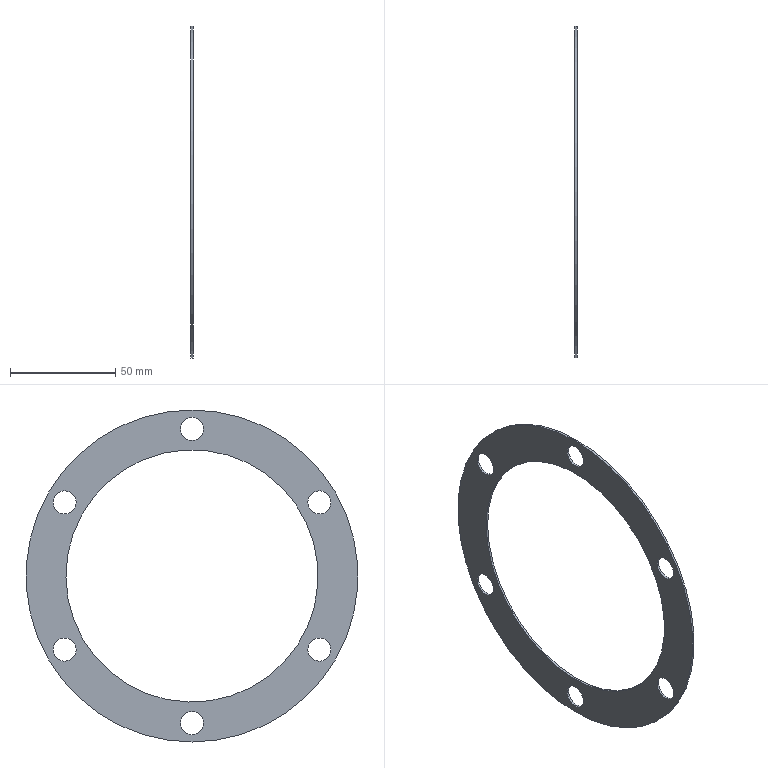Component | NX | T1_GASKET_2 | 1 solid | 10 faces | box 1 x 158 x 158 mm | volume 7727 mm3 | cylinder 8 | plane 2 | commonest cylinder face diameters 11 x6 120 x1 158 x1
STEP:
#1=CARTESIAN_POINT('',(0.,0.,0.));
#2=DIRECTION('',(0.,0.,1.));
#3=DIRECTION('',(1.,0.,0.));
#4=AXIS2_PLACEMENT_3D('',#1,#2,#3);
#5=CARTESIAN_POINT('',(279.,-0.,-78.5));
#6=VERTEX_POINT('',#5);
#7=CARTESIAN_POINT('',(279.,-0.,-73.));
#8=DIRECTION('',(1.,0.,0.));
#9=DIRECTION('',(0.,-0.,-1.));
#10=AXIS2_PLACEMENT_3D('',#7,#8,#9);
#11=CIRCLE('',#10,5.5);
#12=CARTESIAN_POINT('',(279.,-0.,-73.));
#13=DIRECTION('',(-1.,0.,0.));
#14=DIRECTION('',(0.,0.5,0.866));
#15=AXIS2_PLACEMENT_3D('',#12,#13,#14);
#16=CYLINDRICAL_SURFACE('',#15,5.5);
#17=CARTESIAN_POINT('',(8.901,0.));
#18=DIRECTION('',(-1.,0.));
#19=VECTOR('',#18,1.);
#20=LINE('',#17,#19);
#21=(GEOMETRIC_REPRESENTATION_CONTEXT(2)PARAMETRIC_REPRESENTATION_CONTEXT()REPRESENTATION_CONTEXT('',''));
#22=DEFINITIONAL_REPRESENTATION('',(#20),#21);
#23=PCURVE('',#16,#22);
#24=CARTESIAN_POINT('',(279.,30.311,14.5));
#25=DIRECTION('',(1.,0.,0.));
#26=DIRECTION('',(0.,-0.5,-0.866));
#27=AXIS2_PLACEMENT_3D('',#24,#25,#26);
#28=PLANE('',#27);
#29=CARTESIAN_POINT('',(90.933,17.5));
#30=DIRECTION('',(0.866,0.5));
#31=AXIS2_PLACEMENT_2D('',#29,#30);
#32=CIRCLE('',#31,5.5);
#33=(GEOMETRIC_REPRESENTATION_CONTEXT(2)PARAMETRIC_REPRESENTATION_CONTEXT()REPRESENTATION_CONTEXT('',''));
#34=DEFINITIONAL_REPRESENTATION('',(#32),#33);
#35=PCURVE('',#28,#34);
#36=SURFACE_CURVE('',#11,(#23,#35),.PCURVE_S1.);
#37=EDGE_CURVE('',#6,#6,#36,.T.);
#38=ORIENTED_EDGE('',*,*,#37,.F.);
#39=CARTESIAN_POINT('',(278.,-0.,-78.5));
#40=VERTEX_POINT('',#39);
#41=CARTESIAN_POINT('',(279.,-0.,-78.5));
#42=CARTESIAN_POINT('',(278.,-0.,-78.5));
#43=B_SPLINE_CURVE_WITH_KNOTS('',1,(#41,#42),.UNSPECIFIED.,.F.,.F.,(2,2),(0.,1.),.PIECEWISE_BEZIER_KNOTS.);
#44=CARTESIAN_POINT('',(8.901,0.));
#45=DIRECTION('',(0.,1.));
#46=VECTOR('',#45,1.);
#47=LINE('',#44,#46);
#48=(GEOMETRIC_REPRESENTATION_CONTEXT(2)PARAMETRIC_REPRESENTATION_CONTEXT()REPRESENTATION_CONTEXT('',''));
#49=DEFINITIONAL_REPRESENTATION('',(#47),#48);
#50=PCURVE('',#16,#49);
#51=CARTESIAN_POINT('',(2.618,0.));
#52=DIRECTION('',(0.,1.));
#53=VECTOR('',#52,1.);
#54=LINE('',#51,#53);
#55=(GEOMETRIC_REPRESENTATION_CONTEXT(2)PARAMETRIC_REPRESENTATION_CONTEXT()REPRESENTATION_CONTEXT('',''));
#56=DEFINITIONAL_REPRESENTATION('',(#54),#55);
#57=PCURVE('',#16,#56);
#58=SEAM_CURVE('',#43,(#50,#57),.PCURVE_S1.);
#59=EDGE_CURVE('',#6,#40,#58,.T.);
#60=ORIENTED_EDGE('',*,*,#59,.T.);
#61=CARTESIAN_POINT('',(278.,-0.,-73.));
#62=DIRECTION('',(1.,0.,0.));
#63=DIRECTION('',(0.,-0.,-1.));
#64=AXIS2_PLACEMENT_3D('',#61,#62,#63);
#65=CIRCLE('',#64,5.5);
#66=CARTESIAN_POINT('',(8.901,1.));
#67=DIRECTION('',(-1.,0.));
#68=VECTOR('',#67,1.);
#69=LINE('',#66,#68);
#70=(GEOMETRIC_REPRESENTATION_CONTEXT(2)PARAMETRIC_REPRESENTATION_CONTEXT()REPRESENTATION_CONTEXT('',''));
#71=DEFINITIONAL_REPRESENTATION('',(#69),#70);
#72=PCURVE('',#16,#71);
#73=CARTESIAN_POINT('',(278.,30.311,14.5));
#74=DIRECTION('',(1.,0.,0.));
#75=DIRECTION('',(0.,-0.5,-0.866));
#76=AXIS2_PLACEMENT_3D('',#73,#74,#75);
#77=PLANE('',#76);
#78=CARTESIAN_POINT('',(90.933,17.5));
#79=DIRECTION('',(0.866,0.5));
#80=AXIS2_PLACEMENT_2D('',#78,#79);
#81=CIRCLE('',#80,5.5);
#82=(GEOMETRIC_REPRESENTATION_CONTEXT(2)PARAMETRIC_REPRESENTATION_CONTEXT()REPRESENTATION_CONTEXT('',''));
#83=DEFINITIONAL_REPRESENTATION('',(#81),#82);
#84=PCURVE('',#77,#83);
#85=SURFACE_CURVE('',#65,(#72,#84),.PCURVE_S1.);
#86=EDGE_CURVE('',#40,#40,#85,.T.);
#87=ORIENTED_EDGE('',*,*,#86,.T.);
#88=ORIENTED_EDGE('',*,*,#59,.F.);
#89=EDGE_LOOP('',(#38,#60,#87,#88));
#90=FACE_BOUND('',#89,.F.);
#91=ADVANCED_FACE('',(#90),#16,.F.);
#92=CARTESIAN_POINT('',(279.,-65.385,-40.75));
#93=VERTEX_POINT('',#92);
#94=CARTESIAN_POINT('',(279.,-60.622,-38.));
#95=DIRECTION('',(1.,0.,0.));
#96=DIRECTION('',(0.,-0.866,-0.5));
#97=AXIS2_PLACEMENT_3D('',#94,#95,#96);
#98=CIRCLE('',#97,5.5);
#99=CARTESIAN_POINT('',(279.,-60.622,-38.));
#100=DIRECTION('',(-1.,0.,0.));
#101=DIRECTION('',(0.,0.5,0.866));
#102=AXIS2_PLACEMENT_3D('',#99,#100,#101);
#103=CYLINDRICAL_SURFACE('',#102,5.5);
#104=CARTESIAN_POINT('',(9.948,0.));
#105=DIRECTION('',(-1.,0.));
#106=VECTOR('',#105,1.);
#107=LINE('',#104,#106);
#108=(GEOMETRIC_REPRESENTATION_CONTEXT(2)PARAMETRIC_REPRESENTATION_CONTEXT()REPRESENTATION_CONTEXT('',''));
#109=DEFINITIONAL_REPRESENTATION('',(#107),#108);
#110=PCURVE('',#103,#109);
#111=CARTESIAN_POINT('',(90.933,-52.5));
#112=DIRECTION('',(0.866,-0.5));
#113=AXIS2_PLACEMENT_2D('',#111,#112);
#114=CIRCLE('',#113,5.5);
#115=(GEOMETRIC_REPRESENTATION_CONTEXT(2)PARAMETRIC_REPRESENTATION_CONTEXT()REPRESENTATION_CONTEXT('',''));
#116=DEFINITIONAL_REPRESENTATION('',(#114),#115);
#117=PCURVE('',#28,#116);
#118=SURFACE_CURVE('',#98,(#110,#117),.PCURVE_S1.);
#119=EDGE_CURVE('',#93,#93,#118,.T.);
#120=ORIENTED_EDGE('',*,*,#119,.F.);
#121=CARTESIAN_POINT('',(278.,-65.385,-40.75));
#122=VERTEX_POINT('',#121);
#123=CARTESIAN_POINT('',(279.,-65.385,-40.75));
#124=CARTESIAN_POINT('',(278.,-65.385,-40.75));
#125=B_SPLINE_CURVE_WITH_KNOTS('',1,(#123,#124),.UNSPECIFIED.,.F.,.F.,(2,2),(0.,1.),.PIECEWISE_BEZIER_KNOTS.);
#126=CARTESIAN_POINT('',(9.948,0.));
#127=DIRECTION('',(0.,1.));
#128=VECTOR('',#127,1.);
#129=LINE('',#126,#128);
#130=(GEOMETRIC_REPRESENTATION_CONTEXT(2)PARAMETRIC_REPRESENTATION_CONTEXT()REPRESENTATION_CONTEXT('',''));
#131=DEFINITIONAL_REPRESENTATION('',(#129),#130);
#132=PCURVE('',#103,#131);
#133=CARTESIAN_POINT('',(3.665,0.));
#134=DIRECTION('',(0.,1.));
#135=VECTOR('',#134,1.);
#136=LINE('',#133,#135);
#137=(GEOMETRIC_REPRESENTATION_CONTEXT(2)PARAMETRIC_REPRESENTATION_CONTEXT()REPRESENTATION_CONTEXT('',''));
#138=DEFINITIONAL_REPRESENTATION('',(#136),#137);
#139=PCURVE('',#103,#138);
#140=SEAM_CURVE('',#125,(#132,#139),.PCURVE_S1.);
#141=EDGE_CURVE('',#93,#122,#140,.T.);
#142=ORIENTED_EDGE('',*,*,#141,.T.);
#143=CARTESIAN_POINT('',(278.,-60.622,-38.));
#144=DIRECTION('',(1.,0.,0.));
#145=DIRECTION('',(0.,-0.866,-0.5));
#146=AXIS2_PLACEMENT_3D('',#143,#144,#145);
#147=CIRCLE('',#146,5.5);
#148=CARTESIAN_POINT('',(9.948,1.));
#149=DIRECTION('',(-1.,0.));
#150=VECTOR('',#149,1.);
#151=LINE('',#148,#150);
#152=(GEOMETRIC_REPRESENTATION_CONTEXT(2)PARAMETRIC_REPRESENTATION_CONTEXT()REPRESENTATION_CONTEXT('',''));
#153=DEFINITIONAL_REPRESENTATION('',(#151),#152);
#154=PCURVE('',#103,#153);
#155=CARTESIAN_POINT('',(90.933,-52.5));
#156=DIRECTION('',(0.866,-0.5));
#157=AXIS2_PLACEMENT_2D('',#155,#156);
#158=CIRCLE('',#157,5.5);
#159=(GEOMETRIC_REPRESENTATION_CONTEXT(2)PARAMETRIC_REPRESENTATION_CONTEXT()REPRESENTATION_CONTEXT('',''));
#160=DEFINITIONAL_REPRESENTATION('',(#158),#159);
#161=PCURVE('',#77,#160);
#162=SURFACE_CURVE('',#147,(#154,#161),.PCURVE_S1.);
#163=EDGE_CURVE('',#122,#122,#162,.T.);
#164=ORIENTED_EDGE('',*,*,#163,.T.);
#165=ORIENTED_EDGE('',*,*,#141,.F.);
#166=EDGE_LOOP('',(#120,#142,#164,#165));
#167=FACE_BOUND('',#166,.F.);
#168=ADVANCED_FACE('',(#167),#103,.F.);
#169=CARTESIAN_POINT('',(279.,-65.385,34.75));
#170=VERTEX_POINT('',#169);
#171=CARTESIAN_POINT('',(279.,-60.622,32.));
#172=DIRECTION('',(1.,0.,0.));
#173=DIRECTION('',(0.,-0.866,0.5));
#174=AXIS2_PLACEMENT_3D('',#171,#172,#173);
#175=CIRCLE('',#174,5.5);
#176=CARTESIAN_POINT('',(279.,-60.622,32.));
#177=DIRECTION('',(-1.,0.,0.));
#178=DIRECTION('',(0.,0.5,0.866));
#179=AXIS2_PLACEMENT_3D('',#176,#177,#178);
#180=CYLINDRICAL_SURFACE('',#179,5.5);
#181=CARTESIAN_POINT('',(10.996,0.));
#182=DIRECTION('',(-1.,0.));
#183=VECTOR('',#182,1.);
#184=LINE('',#181,#183);
#185=(GEOMETRIC_REPRESENTATION_CONTEXT(2)PARAMETRIC_REPRESENTATION_CONTEXT()REPRESENTATION_CONTEXT('',''));
#186=DEFINITIONAL_REPRESENTATION('',(#184),#185);
#187=PCURVE('',#180,#186);
#188=CARTESIAN_POINT('',(30.311,-87.5));
#189=DIRECTION('',(0.,-1.));
#190=AXIS2_PLACEMENT_2D('',#188,#189);
#191=CIRCLE('',#190,5.5);
#192=(GEOMETRIC_REPRESENTATION_CONTEXT(2)PARAMETRIC_REPRESENTATION_CONTEXT()REPRESENTATION_CONTEXT('',''));
#193=DEFINITIONAL_REPRESENTATION('',(#191),#192);
#194=PCURVE('',#28,#193);
#195=SURFACE_CURVE('',#175,(#187,#194),.PCURVE_S1.);
#196=EDGE_CURVE('',#170,#170,#195,.T.);
#197=ORIENTED_EDGE('',*,*,#196,.F.);
#198=CARTESIAN_POINT('',(278.,-65.385,34.75));
#199=VERTEX_POINT('',#198);
#200=CARTESIAN_POINT('',(279.,-65.385,34.75));
#201=CARTESIAN_POINT('',(278.,-65.385,34.75));
#202=B_SPLINE_CURVE_WITH_KNOTS('',1,(#200,#201),.UNSPECIFIED.,.F.,.F.,(2,2),(0.,1.),.PIECEWISE_BEZIER_KNOTS.);
#203=CARTESIAN_POINT('',(10.996,0.));
#204=DIRECTION('',(0.,1.));
#205=VECTOR('',#204,1.);
#206=LINE('',#203,#205);
#207=(GEOMETRIC_REPRESENTATION_CONTEXT(2)PARAMETRIC_REPRESENTATION_CONTEXT()REPRESENTATION_CONTEXT('',''));
#208=DEFINITIONAL_REPRESENTATION('',(#206),#207);
#209=PCURVE('',#180,#208);
#210=CARTESIAN_POINT('',(4.712,0.));
#211=DIRECTION('',(0.,1.));
#212=VECTOR('',#211,1.);
#213=LINE('',#210,#212);
#214=(GEOMETRIC_REPRESENTATION_CONTEXT(2)PARAMETRIC_REPRESENTATION_CONTEXT()REPRESENTATION_CONTEXT('',''));
#215=DEFINITIONAL_REPRESENTATION('',(#213),#214);
#216=PCURVE('',#180,#215);
#217=SEAM_CURVE('',#202,(#209,#216),.PCURVE_S1.);
#218=EDGE_CURVE('',#170,#199,#217,.T.);
#219=ORIENTED_EDGE('',*,*,#218,.T.);
#220=CARTESIAN_POINT('',(278.,-60.622,32.));
#221=DIRECTION('',(1.,0.,0.));
#222=DIRECTION('',(0.,-0.866,0.5));
#223=AXIS2_PLACEMENT_3D('',#220,#221,#222);
#224=CIRCLE('',#223,5.5);
#225=CARTESIAN_POINT('',(10.996,1.));
#226=DIRECTION('',(-1.,0.));
#227=VECTOR('',#226,1.);
#228=LINE('',#225,#227);
#229=(GEOMETRIC_REPRESENTATION_CONTEXT(2)PARAMETRIC_REPRESENTATION_CONTEXT()REPRESENTATION_CONTEXT('',''));
#230=DEFINITIONAL_REPRESENTATION('',(#228),#229);
#231=PCURVE('',#180,#230);
#232=CARTESIAN_POINT('',(30.311,-87.5));
#233=DIRECTION('',(0.,-1.));
#234=AXIS2_PLACEMENT_2D('',#232,#233);
#235=CIRCLE('',#234,5.5);
#236=(GEOMETRIC_REPRESENTATION_CONTEXT(2)PARAMETRIC_REPRESENTATION_CONTEXT()REPRESENTATION_CONTEXT('',''));
#237=DEFINITIONAL_REPRESENTATION('',(#235),#236);
#238=PCURVE('',#77,#237);
#239=SURFACE_CURVE('',#224,(#231,#238),.PCURVE_S1.);
#240=EDGE_CURVE('',#199,#199,#239,.T.);
#241=ORIENTED_EDGE('',*,*,#240,.T.);
#242=ORIENTED_EDGE('',*,*,#218,.F.);
#243=EDGE_LOOP('',(#197,#219,#241,#242));
#244=FACE_BOUND('',#243,.F.);
#245=ADVANCED_FACE('',(#244),#180,.F.);
#246=CARTESIAN_POINT('',(279.,51.962,-33.));
#247=VERTEX_POINT('',#246);
#248=CARTESIAN_POINT('',(279.,0.,-3.));
#249=DIRECTION('',(1.,0.,0.));
#250=DIRECTION('',(0.,0.866,-0.5));
#251=AXIS2_PLACEMENT_3D('',#248,#249,#250);
#252=CIRCLE('',#251,60.);
#253=CARTESIAN_POINT('',(279.,0.,-3.));
#254=DIRECTION('',(-1.,0.,0.));
#255=DIRECTION('',(0.,0.5,0.866));
#256=AXIS2_PLACEMENT_3D('',#253,#254,#255);
#257=CYLINDRICAL_SURFACE('',#256,60.);
#258=CARTESIAN_POINT('',(7.854,0.));
#259=DIRECTION('',(-1.,0.));
#260=VECTOR('',#259,1.);
#261=LINE('',#258,#260);
#262=(GEOMETRIC_REPRESENTATION_CONTEXT(2)PARAMETRIC_REPRESENTATION_CONTEXT()REPRESENTATION_CONTEXT('',''));
#263=DEFINITIONAL_REPRESENTATION('',(#261),#262);
#264=PCURVE('',#257,#263);
#265=CARTESIAN_POINT('',(30.311,-17.5));
#266=DIRECTION('',(0.,1.));
#267=AXIS2_PLACEMENT_2D('',#265,#266);
#268=CIRCLE('',#267,60.);
#269=(GEOMETRIC_REPRESENTATION_CONTEXT(2)PARAMETRIC_REPRESENTATION_CONTEXT()REPRESENTATION_CONTEXT('',''));
#270=DEFINITIONAL_REPRESENTATION('',(#268),#269);
#271=PCURVE('',#28,#270);
#272=SURFACE_CURVE('',#252,(#264,#271),.PCURVE_S1.);
#273=EDGE_CURVE('',#247,#247,#272,.T.);
#274=ORIENTED_EDGE('',*,*,#273,.F.);
#275=CARTESIAN_POINT('',(278.,51.962,-33.));
#276=VERTEX_POINT('',#275);
#277=CARTESIAN_POINT('',(279.,51.962,-33.));
#278=CARTESIAN_POINT('',(278.,51.962,-33.));
#279=B_SPLINE_CURVE_WITH_KNOTS('',1,(#277,#278),.UNSPECIFIED.,.F.,.F.,(2,2),(0.,1.),.PIECEWISE_BEZIER_KNOTS.);
#280=CARTESIAN_POINT('',(7.854,0.));
#281=DIRECTION('',(0.,1.));
#282=VECTOR('',#281,1.);
#283=LINE('',#280,#282);
#284=(GEOMETRIC_REPRESENTATION_CONTEXT(2)PARAMETRIC_REPRESENTATION_CONTEXT()REPRESENTATION_CONTEXT('',''));
#285=DEFINITIONAL_REPRESENTATION('',(#283),#284);
#286=PCURVE('',#257,#285);
#287=CARTESIAN_POINT('',(1.571,0.));
#288=DIRECTION('',(0.,1.));
#289=VECTOR('',#288,1.);
#290=LINE('',#287,#289);
#291=(GEOMETRIC_REPRESENTATION_CONTEXT(2)PARAMETRIC_REPRESENTATION_CONTEXT()REPRESENTATION_CONTEXT('',''));
#292=DEFINITIONAL_REPRESENTATION('',(#290),#291);
#293=PCURVE('',#257,#292);
#294=SEAM_CURVE('',#279,(#286,#293),.PCURVE_S1.);
#295=EDGE_CURVE('',#247,#276,#294,.T.);
#296=ORIENTED_EDGE('',*,*,#295,.T.);
#297=CARTESIAN_POINT('',(278.,0.,-3.));
#298=DIRECTION('',(1.,0.,0.));
#299=DIRECTION('',(0.,0.866,-0.5));
#300=AXIS2_PLACEMENT_3D('',#297,#298,#299);
#301=CIRCLE('',#300,60.);
#302=CARTESIAN_POINT('',(7.854,1.));
#303=DIRECTION('',(-1.,0.));
#304=VECTOR('',#303,1.);
#305=LINE('',#302,#304);
#306=(GEOMETRIC_REPRESENTATION_CONTEXT(2)PARAMETRIC_REPRESENTATION_CONTEXT()REPRESENTATION_CONTEXT('',''));
#307=DEFINITIONAL_REPRESENTATION('',(#305),#306);
#308=PCURVE('',#257,#307);
#309=CARTESIAN_POINT('',(30.311,-17.5));
#310=DIRECTION('',(0.,1.));
#311=AXIS2_PLACEMENT_2D('',#309,#310);
#312=CIRCLE('',#311,60.);
#313=(GEOMETRIC_REPRESENTATION_CONTEXT(2)PARAMETRIC_REPRESENTATION_CONTEXT()REPRESENTATION_CONTEXT('',''));
#314=DEFINITIONAL_REPRESENTATION('',(#312),#313);
#315=PCURVE('',#77,#314);
#316=SURFACE_CURVE('',#301,(#308,#315),.PCURVE_S1.);
#317=EDGE_CURVE('',#276,#276,#316,.T.);
#318=ORIENTED_EDGE('',*,*,#317,.T.);
#319=ORIENTED_EDGE('',*,*,#295,.F.);
#320=EDGE_LOOP('',(#274,#296,#318,#319));
#321=FACE_BOUND('',#320,.F.);
#322=ADVANCED_FACE('',(#321),#257,.F.);
#323=CARTESIAN_POINT('',(279.,0.,72.5));
#324=VERTEX_POINT('',#323);
#325=CARTESIAN_POINT('',(279.,0.,67.));
#326=DIRECTION('',(1.,0.,0.));
#327=DIRECTION('',(0.,0.,1.));
#328=AXIS2_PLACEMENT_3D('',#325,#326,#327);
#329=CIRCLE('',#328,5.5);
#330=CARTESIAN_POINT('',(279.,0.,67.));
#331=DIRECTION('',(-1.,0.,0.));
#332=DIRECTION('',(0.,0.5,0.866));
#333=AXIS2_PLACEMENT_3D('',#330,#331,#332);
#334=CYLINDRICAL_SURFACE('',#333,5.5);
#335=CARTESIAN_POINT('',(12.043,0.));
#336=DIRECTION('',(-1.,0.));
#337=VECTOR('',#336,1.);
#338=LINE('',#335,#337);
#339=(GEOMETRIC_REPRESENTATION_CONTEXT(2)PARAMETRIC_REPRESENTATION_CONTEXT()REPRESENTATION_CONTEXT('',''));
#340=DEFINITIONAL_REPRESENTATION('',(#338),#339);
#341=PCURVE('',#334,#340);
#342=CARTESIAN_POINT('',(-30.311,-52.5));
#343=DIRECTION('',(-0.866,-0.5));
#344=AXIS2_PLACEMENT_2D('',#342,#343);
#345=CIRCLE('',#344,5.5);
#346=(GEOMETRIC_REPRESENTATION_CONTEXT(2)PARAMETRIC_REPRESENTATION_CONTEXT()REPRESENTATION_CONTEXT('',''));
#347=DEFINITIONAL_REPRESENTATION('',(#345),#346);
#348=PCURVE('',#28,#347);
#349=SURFACE_CURVE('',#329,(#341,#348),.PCURVE_S1.);
#350=EDGE_CURVE('',#324,#324,#349,.T.);
#351=ORIENTED_EDGE('',*,*,#350,.F.);
#352=CARTESIAN_POINT('',(278.,0.,72.5));
#353=VERTEX_POINT('',#352);
#354=CARTESIAN_POINT('',(279.,0.,72.5));
#355=CARTESIAN_POINT('',(278.,0.,72.5));
#356=B_SPLINE_CURVE_WITH_KNOTS('',1,(#354,#355),.UNSPECIFIED.,.F.,.F.,(2,2),(0.,1.),.PIECEWISE_BEZIER_KNOTS.);
#357=CARTESIAN_POINT('',(12.043,0.));
#358=DIRECTION('',(0.,1.));
#359=VECTOR('',#358,1.);
#360=LINE('',#357,#359);
#361=(GEOMETRIC_REPRESENTATION_CONTEXT(2)PARAMETRIC_REPRESENTATION_CONTEXT()REPRESENTATION_CONTEXT('',''));
#362=DEFINITIONAL_REPRESENTATION('',(#360),#361);
#363=PCURVE('',#334,#362);
#364=CARTESIAN_POINT('',(5.76,0.));
#365=DIRECTION('',(0.,1.));
#366=VECTOR('',#365,1.);
#367=LINE('',#364,#366);
#368=(GEOMETRIC_REPRESENTATION_CONTEXT(2)PARAMETRIC_REPRESENTATION_CONTEXT()REPRESENTATION_CONTEXT('',''));
#369=DEFINITIONAL_REPRESENTATION('',(#367),#368);
#370=PCURVE('',#334,#369);
#371=SEAM_CURVE('',#356,(#363,#370),.PCURVE_S1.);
#372=EDGE_CURVE('',#324,#353,#371,.T.);
#373=ORIENTED_EDGE('',*,*,#372,.T.);
#374=CARTESIAN_POINT('',(278.,0.,67.));
#375=DIRECTION('',(1.,0.,0.));
#376=DIRECTION('',(0.,0.,1.));
#377=AXIS2_PLACEMENT_3D('',#374,#375,#376);
#378=CIRCLE('',#377,5.5);
#379=CARTESIAN_POINT('',(12.043,1.));
#380=DIRECTION('',(-1.,0.));
#381=VECTOR('',#380,1.);
#382=LINE('',#379,#381);
#383=(GEOMETRIC_REPRESENTATION_CONTEXT(2)PARAMETRIC_REPRESENTATION_CONTEXT()REPRESENTATION_CONTEXT('',''));
#384=DEFINITIONAL_REPRESENTATION('',(#382),#383);
#385=PCURVE('',#334,#384);
#386=CARTESIAN_POINT('',(-30.311,-52.5));
#387=DIRECTION('',(-0.866,-0.5));
#388=AXIS2_PLACEMENT_2D('',#386,#387);
#389=CIRCLE('',#388,5.5);
#390=(GEOMETRIC_REPRESENTATION_CONTEXT(2)PARAMETRIC_REPRESENTATION_CONTEXT()REPRESENTATION_CONTEXT('',''));
#391=DEFINITIONAL_REPRESENTATION('',(#389),#390);
#392=PCURVE('',#77,#391);
#393=SURFACE_CURVE('',#378,(#385,#392),.PCURVE_S1.);
#394=EDGE_CURVE('',#353,#353,#393,.T.);
#395=ORIENTED_EDGE('',*,*,#394,.T.);
#396=ORIENTED_EDGE('',*,*,#372,.F.);
#397=EDGE_LOOP('',(#351,#373,#395,#396));
#398=FACE_BOUND('',#397,.F.);
#399=ADVANCED_FACE('',(#398),#334,.F.);
#400=CARTESIAN_POINT('',(279.,65.385,34.75));
#401=VERTEX_POINT('',#400);
#402=CARTESIAN_POINT('',(279.,60.622,32.));
#403=DIRECTION('',(1.,0.,0.));
#404=DIRECTION('',(0.,0.866,0.5));
#405=AXIS2_PLACEMENT_3D('',#402,#403,#404);
#406=CIRCLE('',#405,5.5);
#407=CARTESIAN_POINT('',(279.,60.622,32.));
#408=DIRECTION('',(-1.,0.,0.));
#409=DIRECTION('',(0.,0.5,0.866));
#410=AXIS2_PLACEMENT_3D('',#407,#408,#409);
#411=CYLINDRICAL_SURFACE('',#410,5.5);
#412=CARTESIAN_POINT('',(6.807,0.));
#413=DIRECTION('',(-1.,0.));
#414=VECTOR('',#413,1.);
#415=LINE('',#412,#414);
#416=(GEOMETRIC_REPRESENTATION_CONTEXT(2)PARAMETRIC_REPRESENTATION_CONTEXT()REPRESENTATION_CONTEXT('',''));
#417=DEFINITIONAL_REPRESENTATION('',(#415),#416);
#418=PCURVE('',#411,#417);
#419=CARTESIAN_POINT('',(-30.311,17.5));
#420=DIRECTION('',(-0.866,0.5));
#421=AXIS2_PLACEMENT_2D('',#419,#420);
#422=CIRCLE('',#421,5.5);
#423=(GEOMETRIC_REPRESENTATION_CONTEXT(2)PARAMETRIC_REPRESENTATION_CONTEXT()REPRESENTATION_CONTEXT('',''));
#424=DEFINITIONAL_REPRESENTATION('',(#422),#423);
#425=PCURVE('',#28,#424);
#426=SURFACE_CURVE('',#406,(#418,#425),.PCURVE_S1.);
#427=EDGE_CURVE('',#401,#401,#426,.T.);
#428=ORIENTED_EDGE('',*,*,#427,.F.);
#429=CARTESIAN_POINT('',(278.,65.385,34.75));
#430=VERTEX_POINT('',#429);
#431=CARTESIAN_POINT('',(279.,65.385,34.75));
#432=CARTESIAN_POINT('',(278.,65.385,34.75));
#433=B_SPLINE_CURVE_WITH_KNOTS('',1,(#431,#432),.UNSPECIFIED.,.F.,.F.,(2,2),(0.,1.),.PIECEWISE_BEZIER_KNOTS.);
#434=CARTESIAN_POINT('',(6.807,0.));
#435=DIRECTION('',(0.,1.));
#436=VECTOR('',#435,1.);
#437=LINE('',#434,#436);
#438=(GEOMETRIC_REPRESENTATION_CONTEXT(2)PARAMETRIC_REPRESENTATION_CONTEXT()REPRESENTATION_CONTEXT('',''));
#439=DEFINITIONAL_REPRESENTATION('',(#437),#438);
#440=PCURVE('',#411,#439);
#441=CARTESIAN_POINT('',(0.5236,0.));
#442=DIRECTION('',(0.,1.));
#443=VECTOR('',#442,1.);
#444=LINE('',#441,#443);
#445=(GEOMETRIC_REPRESENTATION_CONTEXT(2)PARAMETRIC_REPRESENTATION_CONTEXT()REPRESENTATION_CONTEXT('',''));
#446=DEFINITIONAL_REPRESENTATION('',(#444),#445);
#447=PCURVE('',#411,#446);
#448=SEAM_CURVE('',#433,(#440,#447),.PCURVE_S1.);
#449=EDGE_CURVE('',#401,#430,#448,.T.);
#450=ORIENTED_EDGE('',*,*,#449,.T.);
#451=CARTESIAN_POINT('',(278.,60.622,32.));
#452=DIRECTION('',(1.,0.,0.));
#453=DIRECTION('',(0.,0.866,0.5));
#454=AXIS2_PLACEMENT_3D('',#451,#452,#453);
#455=CIRCLE('',#454,5.5);
#456=CARTESIAN_POINT('',(6.807,1.));
#457=DIRECTION('',(-1.,0.));
#458=VECTOR('',#457,1.);
#459=LINE('',#456,#458);
#460=(GEOMETRIC_REPRESENTATION_CONTEXT(2)PARAMETRIC_REPRESENTATION_CONTEXT()REPRESENTATION_CONTEXT('',''));
#461=DEFINITIONAL_REPRESENTATION('',(#459),#460);
#462=PCURVE('',#411,#461);
#463=CARTESIAN_POINT('',(-30.311,17.5));
#464=DIRECTION('',(-0.866,0.5));
#465=AXIS2_PLACEMENT_2D('',#463,#464);
#466=CIRCLE('',#465,5.5);
#467=(GEOMETRIC_REPRESENTATION_CONTEXT(2)PARAMETRIC_REPRESENTATION_CONTEXT()REPRESENTATION_CONTEXT('',''));
#468=DEFINITIONAL_REPRESENTATION('',(#466),#467);
#469=PCURVE('',#77,#468);
#470=SURFACE_CURVE('',#455,(#462,#469),.PCURVE_S1.);
#471=EDGE_CURVE('',#430,#430,#470,.T.);
#472=ORIENTED_EDGE('',*,*,#471,.T.);
#473=ORIENTED_EDGE('',*,*,#449,.F.);
#474=EDGE_LOOP('',(#428,#450,#472,#473));
#475=FACE_BOUND('',#474,.F.);
#476=ADVANCED_FACE('',(#475),#411,.F.);
#477=CARTESIAN_POINT('',(279.,68.416,-42.5));
#478=VERTEX_POINT('',#477);
#479=CARTESIAN_POINT('',(279.,0.,-3.));
#480=DIRECTION('',(1.,0.,0.));
#481=DIRECTION('',(0.,0.866,-0.5));
#482=AXIS2_PLACEMENT_3D('',#479,#480,#481);
#483=CIRCLE('',#482,79.);
#484=CARTESIAN_POINT('',(279.,0.,-3.));
#485=DIRECTION('',(-1.,0.,0.));
#486=DIRECTION('',(0.,0.5,0.866));
#487=AXIS2_PLACEMENT_3D('',#484,#485,#486);
#488=CYLINDRICAL_SURFACE('',#487,79.);
#489=CARTESIAN_POINT('',(7.854,0.));
#490=DIRECTION('',(-1.,0.));
#491=VECTOR('',#490,1.);
#492=LINE('',#489,#491);
#493=(GEOMETRIC_REPRESENTATION_CONTEXT(2)PARAMETRIC_REPRESENTATION_CONTEXT()REPRESENTATION_CONTEXT('',''));
#494=DEFINITIONAL_REPRESENTATION('',(#492),#493);
#495=PCURVE('',#488,#494);
#496=CARTESIAN_POINT('',(30.311,-17.5));
#497=DIRECTION('',(0.,1.));
#498=AXIS2_PLACEMENT_2D('',#496,#497);
#499=CIRCLE('',#498,79.);
#500=(GEOMETRIC_REPRESENTATION_CONTEXT(2)PARAMETRIC_REPRESENTATION_CONTEXT()REPRESENTATION_CONTEXT('',''));
#501=DEFINITIONAL_REPRESENTATION('',(#499),#500);
#502=PCURVE('',#28,#501);
#503=SURFACE_CURVE('',#483,(#495,#502),.PCURVE_S1.);
#504=EDGE_CURVE('',#478,#478,#503,.T.);
#505=ORIENTED_EDGE('',*,*,#504,.F.);
#506=CARTESIAN_POINT('',(278.,68.416,-42.5));
#507=VERTEX_POINT('',#506);
#508=CARTESIAN_POINT('',(279.,68.416,-42.5));
#509=CARTESIAN_POINT('',(278.,68.416,-42.5));
#510=B_SPLINE_CURVE_WITH_KNOTS('',1,(#508,#509),.UNSPECIFIED.,.F.,.F.,(2,2),(0.,1.),.PIECEWISE_BEZIER_KNOTS.);
#511=CARTESIAN_POINT('',(7.854,0.));
#512=DIRECTION('',(0.,1.));
#513=VECTOR('',#512,1.);
#514=LINE('',#511,#513);
#515=(GEOMETRIC_REPRESENTATION_CONTEXT(2)PARAMETRIC_REPRESENTATION_CONTEXT()REPRESENTATION_CONTEXT('',''));
#516=DEFINITIONAL_REPRESENTATION('',(#514),#515);
#517=PCURVE('',#488,#516);
#518=CARTESIAN_POINT('',(1.571,0.));
#519=DIRECTION('',(0.,1.));
#520=VECTOR('',#519,1.);
#521=LINE('',#518,#520);
#522=(GEOMETRIC_REPRESENTATION_CONTEXT(2)PARAMETRIC_REPRESENTATION_CONTEXT()REPRESENTATION_CONTEXT('',''));
#523=DEFINITIONAL_REPRESENTATION('',(#521),#522);
#524=PCURVE('',#488,#523);
#525=SEAM_CURVE('',#510,(#517,#524),.PCURVE_S1.);
#526=EDGE_CURVE('',#478,#507,#525,.T.);
#527=ORIENTED_EDGE('',*,*,#526,.T.);
#528=CARTESIAN_POINT('',(278.,0.,-3.));
#529=DIRECTION('',(1.,0.,0.));
#530=DIRECTION('',(0.,0.866,-0.5));
#531=AXIS2_PLACEMENT_3D('',#528,#529,#530);
#532=CIRCLE('',#531,79.);
#533=CARTESIAN_POINT('',(7.854,1.));
#534=DIRECTION('',(-1.,0.));
#535=VECTOR('',#534,1.);
#536=LINE('',#533,#535);
#537=(GEOMETRIC_REPRESENTATION_CONTEXT(2)PARAMETRIC_REPRESENTATION_CONTEXT()REPRESENTATION_CONTEXT('',''));
#538=DEFINITIONAL_REPRESENTATION('',(#536),#537);
#539=PCURVE('',#488,#538);
#540=CARTESIAN_POINT('',(30.311,-17.5));
#541=DIRECTION('',(0.,1.));
#542=AXIS2_PLACEMENT_2D('',#540,#541);
#543=CIRCLE('',#542,79.);
#544=(GEOMETRIC_REPRESENTATION_CONTEXT(2)PARAMETRIC_REPRESENTATION_CONTEXT()REPRESENTATION_CONTEXT('',''));
#545=DEFINITIONAL_REPRESENTATION('',(#543),#544);
#546=PCURVE('',#77,#545);
#547=SURFACE_CURVE('',#532,(#539,#546),.PCURVE_S1.);
#548=EDGE_CURVE('',#507,#507,#547,.T.);
#549=ORIENTED_EDGE('',*,*,#548,.T.);
#550=ORIENTED_EDGE('',*,*,#526,.F.);
#551=EDGE_LOOP('',(#505,#527,#549,#550));
#552=FACE_BOUND('',#551,.T.);
#553=ADVANCED_FACE('',(#552),#488,.T.);
#554=CARTESIAN_POINT('',(279.,65.385,-40.75));
#555=VERTEX_POINT('',#554);
#556=CARTESIAN_POINT('',(279.,60.622,-38.));
#557=DIRECTION('',(1.,0.,0.));
#558=DIRECTION('',(0.,0.866,-0.5));
#559=AXIS2_PLACEMENT_3D('',#556,#557,#558);
#560=CIRCLE('',#559,5.5);
#561=CARTESIAN_POINT('',(279.,60.622,-38.));
#562=DIRECTION('',(-1.,0.,0.));
#563=DIRECTION('',(0.,0.5,0.866));
#564=AXIS2_PLACEMENT_3D('',#561,#562,#563);
#565=CYLINDRICAL_SURFACE('',#564,5.5);
#566=CARTESIAN_POINT('',(7.854,0.));
#567=DIRECTION('',(-1.,0.));
#568=VECTOR('',#567,1.);
#569=LINE('',#566,#568);
#570=(GEOMETRIC_REPRESENTATION_CONTEXT(2)PARAMETRIC_REPRESENTATION_CONTEXT()REPRESENTATION_CONTEXT('',''));
#571=DEFINITIONAL_REPRESENTATION('',(#569),#570);
#572=PCURVE('',#565,#571);
#573=CARTESIAN_POINT('',(30.311,52.5));
#574=DIRECTION('',(-0.,1.));
#575=AXIS2_PLACEMENT_2D('',#573,#574);
#576=CIRCLE('',#575,5.5);
#577=(GEOMETRIC_REPRESENTATION_CONTEXT(2)PARAMETRIC_REPRESENTATION_CONTEXT()REPRESENTATION_CONTEXT('',''));
#578=DEFINITIONAL_REPRESENTATION('',(#576),#577);
#579=PCURVE('',#28,#578);
#580=SURFACE_CURVE('',#560,(#572,#579),.PCURVE_S1.);
#581=EDGE_CURVE('',#555,#555,#580,.T.);
#582=ORIENTED_EDGE('',*,*,#581,.F.);
#583=CARTESIAN_POINT('',(278.,65.385,-40.75));
#584=VERTEX_POINT('',#583);
#585=CARTESIAN_POINT('',(279.,65.385,-40.75));
#586=CARTESIAN_POINT('',(278.,65.385,-40.75));
#587=B_SPLINE_CURVE_WITH_KNOTS('',1,(#585,#586),.UNSPECIFIED.,.F.,.F.,(2,2),(0.,1.),.PIECEWISE_BEZIER_KNOTS.);
#588=CARTESIAN_POINT('',(7.854,0.));
#589=DIRECTION('',(0.,1.));
#590=VECTOR('',#589,1.);
#591=LINE('',#588,#590);
#592=(GEOMETRIC_REPRESENTATION_CONTEXT(2)PARAMETRIC_REPRESENTATION_CONTEXT()REPRESENTATION_CONTEXT('',''));
#593=DEFINITIONAL_REPRESENTATION('',(#591),#592);
#594=PCURVE('',#565,#593);
#595=CARTESIAN_POINT('',(1.571,0.));
#596=DIRECTION('',(0.,1.));
#597=VECTOR('',#596,1.);
#598=LINE('',#595,#597);
#599=(GEOMETRIC_REPRESENTATION_CONTEXT(2)PARAMETRIC_REPRESENTATION_CONTEXT()REPRESENTATION_CONTEXT('',''));
#600=DEFINITIONAL_REPRESENTATION('',(#598),#599);
#601=PCURVE('',#565,#600);
#602=SEAM_CURVE('',#587,(#594,#601),.PCURVE_S1.);
#603=EDGE_CURVE('',#555,#584,#602,.T.);
#604=ORIENTED_EDGE('',*,*,#603,.T.);
#605=CARTESIAN_POINT('',(278.,60.622,-38.));
#606=DIRECTION('',(1.,0.,0.));
#607=DIRECTION('',(0.,0.866,-0.5));
#608=AXIS2_PLACEMENT_3D('',#605,#606,#607);
#609=CIRCLE('',#608,5.5);
#610=CARTESIAN_POINT('',(7.854,1.));
#611=DIRECTION('',(-1.,0.));
#612=VECTOR('',#611,1.);
#613=LINE('',#610,#612);
#614=(GEOMETRIC_REPRESENTATION_CONTEXT(2)PARAMETRIC_REPRESENTATION_CONTEXT()REPRESENTATION_CONTEXT('',''));
#615=DEFINITIONAL_REPRESENTATION('',(#613),#614);
#616=PCURVE('',#565,#615);
#617=CARTESIAN_POINT('',(30.311,52.5));
#618=DIRECTION('',(-0.,1.));
#619=AXIS2_PLACEMENT_2D('',#617,#618);
#620=CIRCLE('',#619,5.5);
#621=(GEOMETRIC_REPRESENTATION_CONTEXT(2)PARAMETRIC_REPRESENTATION_CONTEXT()REPRESENTATION_CONTEXT('',''));
#622=DEFINITIONAL_REPRESENTATION('',(#620),#621);
#623=PCURVE('',#77,#622);
#624=SURFACE_CURVE('',#609,(#616,#623),.PCURVE_S1.);
#625=EDGE_CURVE('',#584,#584,#624,.T.);
#626=ORIENTED_EDGE('',*,*,#625,.T.);
#627=ORIENTED_EDGE('',*,*,#603,.F.);
#628=EDGE_LOOP('',(#582,#604,#626,#627));
#629=FACE_BOUND('',#628,.F.);
#630=ADVANCED_FACE('',(#629),#565,.F.);
#631=ORIENTED_EDGE('',*,*,#504,.T.);
#632=EDGE_LOOP('',(#631));
#633=FACE_BOUND('',#632,.T.);
#634=ORIENTED_EDGE('',*,*,#427,.F.);
#635=EDGE_LOOP('',(#634));
#636=FACE_BOUND('',#635,.T.);
#637=ORIENTED_EDGE('',*,*,#350,.F.);
#638=EDGE_LOOP('',(#637));
#639=FACE_BOUND('',#638,.T.);
#640=ORIENTED_EDGE('',*,*,#273,.F.);
#641=EDGE_LOOP('',(#640));
#642=FACE_BOUND('',#641,.T.);
#643=ORIENTED_EDGE('',*,*,#196,.F.);
#644=EDGE_LOOP('',(#643));
#645=FACE_BOUND('',#644,.T.);
#646=ORIENTED_EDGE('',*,*,#119,.F.);
#647=EDGE_LOOP('',(#646));
#648=FACE_BOUND('',#647,.T.);
#649=ORIENTED_EDGE('',*,*,#37,.F.);
#650=EDGE_LOOP('',(#649));
#651=FACE_BOUND('',#650,.T.);
#652=ORIENTED_EDGE('',*,*,#581,.F.);
#653=EDGE_LOOP('',(#652));
#654=FACE_BOUND('',#653,.T.);
#655=ADVANCED_FACE('',(#633,#636,#639,#642,#645,#648,#651,#654),#28,.T.);
#656=ORIENTED_EDGE('',*,*,#548,.F.);
#657=EDGE_LOOP('',(#656));
#658=FACE_BOUND('',#657,.T.);
#659=ORIENTED_EDGE('',*,*,#471,.T.);
#660=EDGE_LOOP('',(#659));
#661=FACE_BOUND('',#660,.T.);
#662=ORIENTED_EDGE('',*,*,#394,.T.);
#663=EDGE_LOOP('',(#662));
#664=FACE_BOUND('',#663,.T.);
#665=ORIENTED_EDGE('',*,*,#317,.T.);
#666=EDGE_LOOP('',(#665));
#667=FACE_BOUND('',#666,.T.);
#668=ORIENTED_EDGE('',*,*,#240,.T.);
#669=EDGE_LOOP('',(#668));
#670=FACE_BOUND('',#669,.T.);
#671=ORIENTED_EDGE('',*,*,#163,.T.);
#672=EDGE_LOOP('',(#671));
#673=FACE_BOUND('',#672,.T.);
#674=ORIENTED_EDGE('',*,*,#86,.T.);
#675=EDGE_LOOP('',(#674));
#676=FACE_BOUND('',#675,.T.);
#677=ORIENTED_EDGE('',*,*,#625,.T.);
#678=EDGE_LOOP('',(#677));
#679=FACE_BOUND('',#678,.T.);
#680=ADVANCED_FACE('',(#658,#661,#664,#667,#670,#673,#676,#679),#77,.F.);
#681=CLOSED_SHELL('',(#91,#168,#245,#322,#399,#476,#553,#630,#655,#680));
#682=MANIFOLD_SOLID_BREP('',#681);
#683=(LENGTH_UNIT()NAMED_UNIT(*)SI_UNIT(.MILLI.,.METRE.));
#684=UNCERTAINTY_MEASURE_WITH_UNIT(LENGTH_MEASURE(0.00001),#683,'','');
#685=(NAMED_UNIT(*)PLANE_ANGLE_UNIT()SI_UNIT($,.RADIAN.));
#686=(NAMED_UNIT(*)SI_UNIT($,.STERADIAN.)SOLID_ANGLE_UNIT());
#687=(GEOMETRIC_REPRESENTATION_CONTEXT(3)GLOBAL_UNCERTAINTY_ASSIGNED_CONTEXT((#684))GLOBAL_UNIT_ASSIGNED_CONTEXT((#683,#685,#686))REPRESENTATION_CONTEXT('',''));
#688=ADVANCED_BREP_SHAPE_REPRESENTATION('',(#4,#682),#687);